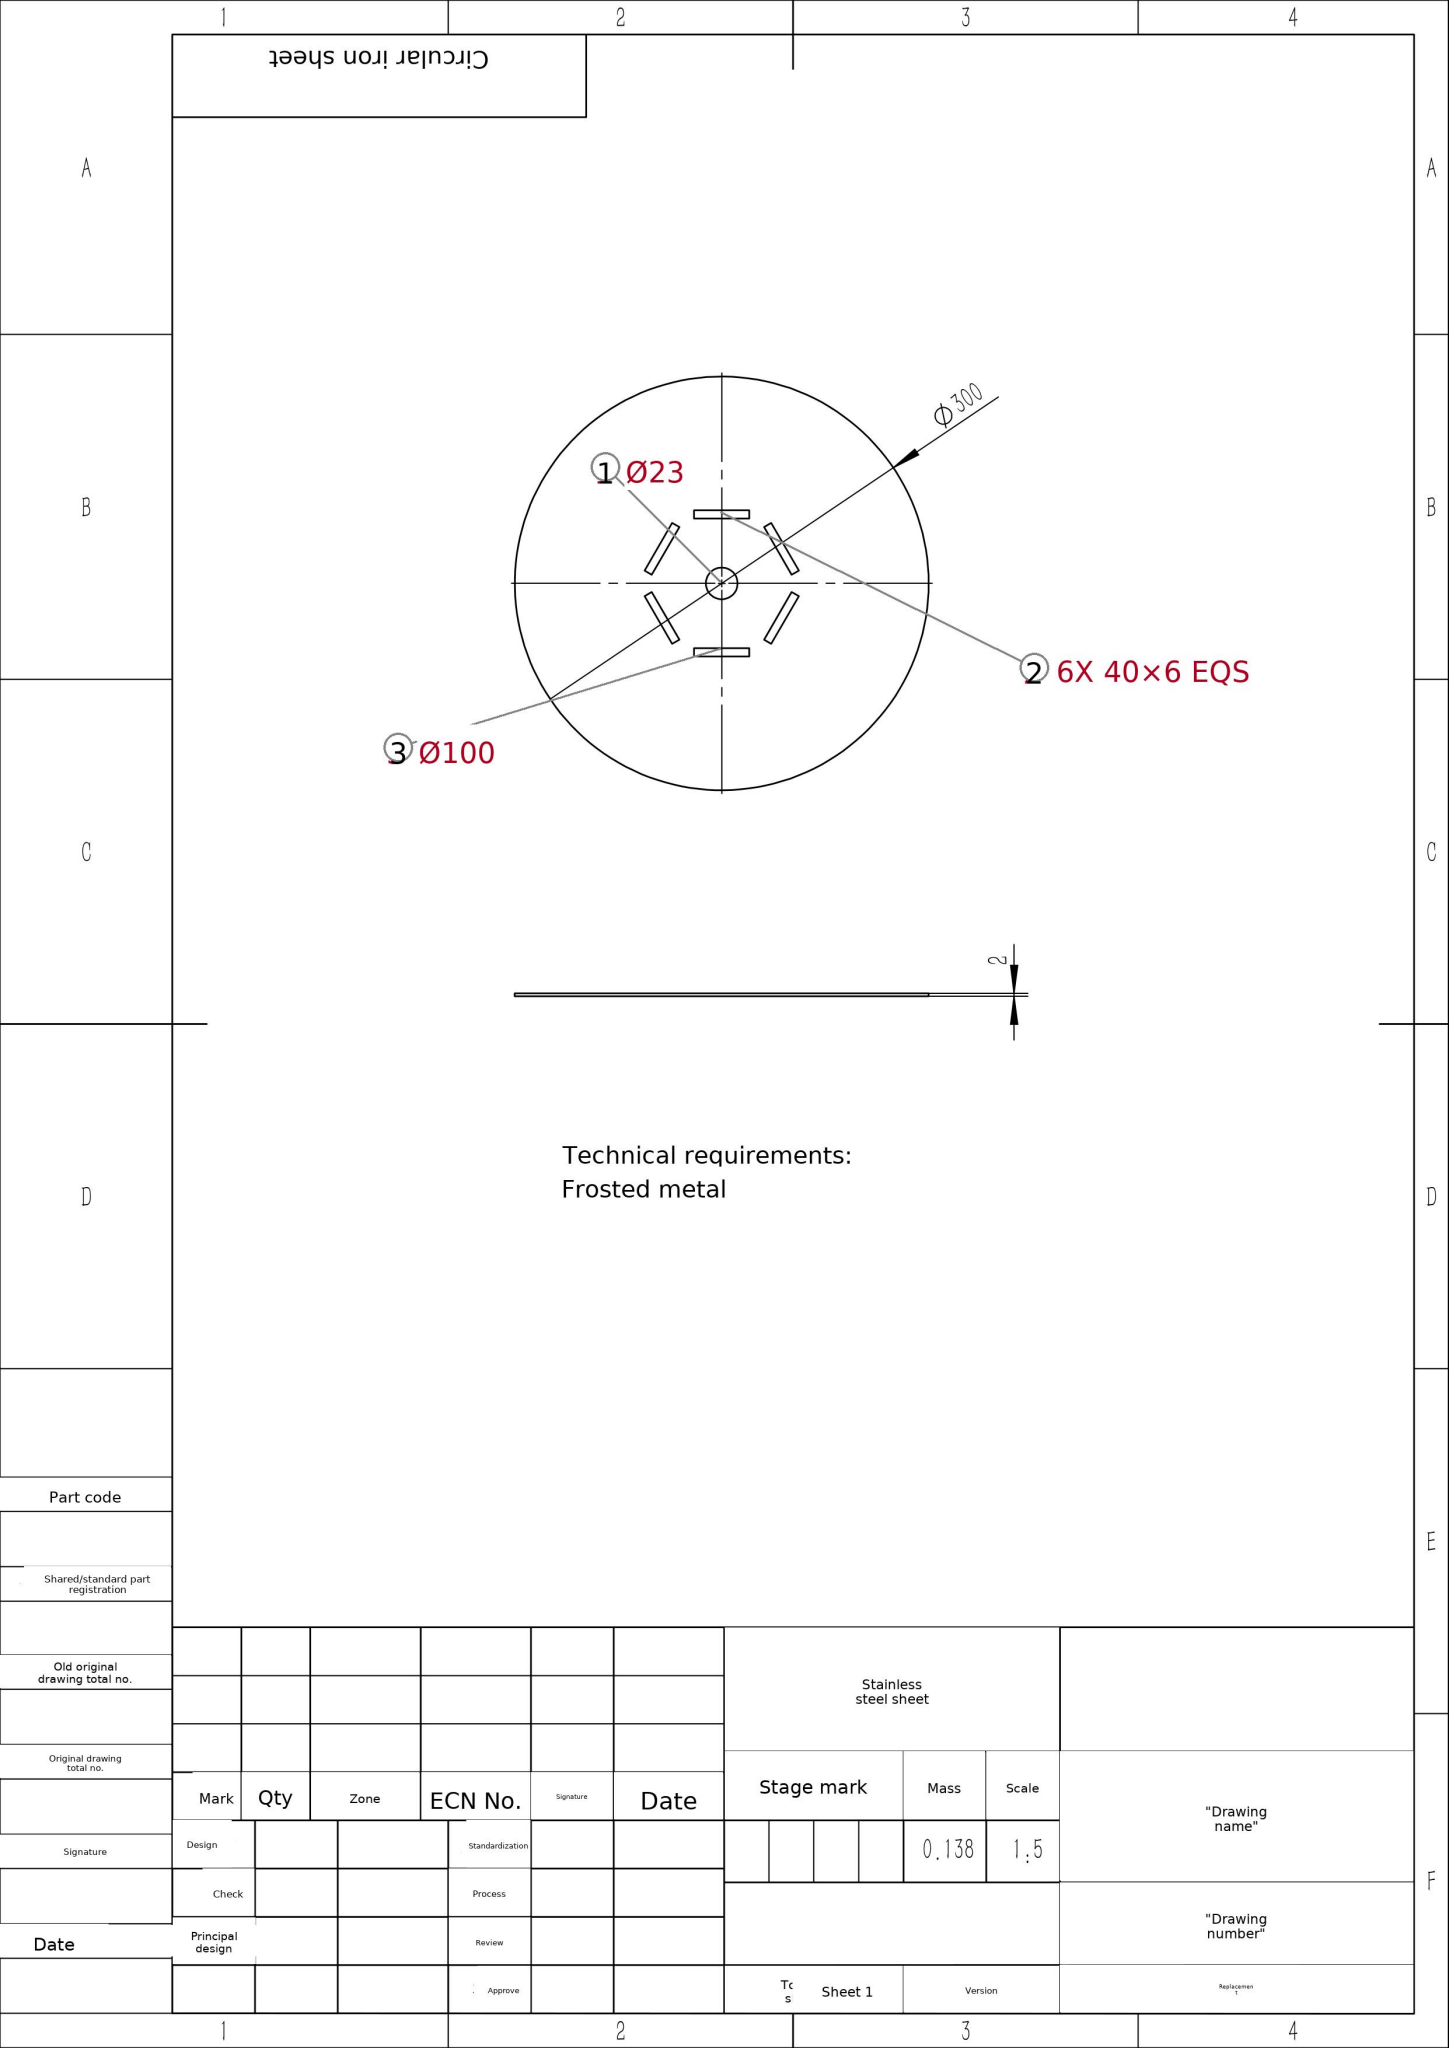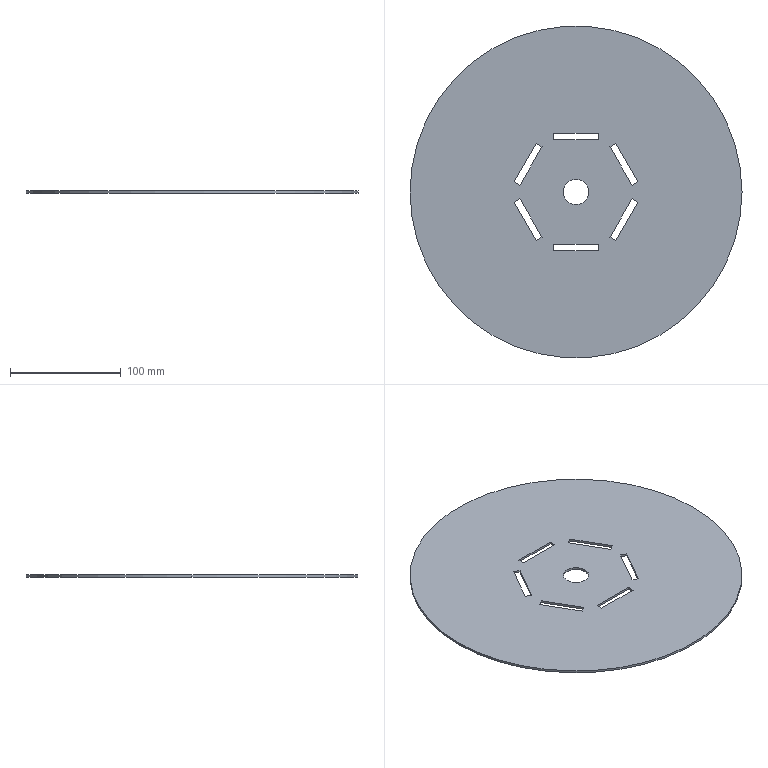Part | SolidWorks | mm | material Stainless steel sheet | 1 solid | 30 faces | box 300 x 300 x 2 mm | volume 137661 mm3 | plane 26 | cylinder 4 | commonest cylinder face diameters 23 x2 300 x2
build123d program:
from build123d import *

# Parameters (mm, degrees)
SKETCH1_R           = 150
SKETCH1_R_2         = 11.5
BOSS_EXTRUDE1_DEPTH = 2
SKETCH3_W           = 40
SKETCH3_H           = 6
CUT_EXTRUDE1_DEPTH  = 2
CIRPATTERN1_COUNT   = 6


with BuildPart() as part:
    # Sketch1 → Boss-Extrude1 (new body)
    with BuildSketch(Plane.XY):
        Circle(SKETCH1_R)
        Circle(SKETCH1_R_2, mode=Mode.SUBTRACT)
    extrude(amount=BOSS_EXTRUDE1_DEPTH)

    # Sketch3 → Cut-Extrude1 (cut)
    with BuildSketch(Plane.XY.offset(2)):
        with Locations((0, 50)):
            Rectangle(SKETCH3_W, SKETCH3_H)
    cut_extrude1 = extrude(amount=-CUT_EXTRUDE1_DEPTH, mode=Mode.SUBTRACT)

    # CirPattern1: Cut-Extrude1 ×6 about axis
    cirpattern1_axis = Axis((0, 0, 0), (0, 0, 1))
    for i in range(1, CIRPATTERN1_COUNT):
        add(cut_extrude1.rotate(cirpattern1_axis, i * 360 / CIRPATTERN1_COUNT), mode=Mode.SUBTRACT)


solid = part.part
STEP:
#1=CARTESIAN_POINT('',(-11.5,0.,2.));
#2=VERTEX_POINT('',#1);
#3=CARTESIAN_POINT('',(11.5,0.,2.));
#4=VERTEX_POINT('',#3);
#5=CARTESIAN_POINT('',(0.,0.,2.));
#6=DIRECTION('',(0.,0.,1.));
#7=DIRECTION('',(1.,0.,0.));
#8=AXIS2_PLACEMENT_3D('',#5,#6,#7);
#9=CIRCLE('',#8,11.5);
#10=EDGE_CURVE('',#2,#4,#9,.T.);
#11=ORIENTED_EDGE('',*,*,#10,.T.);
#12=CARTESIAN_POINT('',(11.5,0.,0.));
#13=VERTEX_POINT('',#12);
#14=CARTESIAN_POINT('',(11.5,0.,2.));
#15=DIRECTION('',(0.,0.,-1.));
#16=VECTOR('',#15,1000.);
#17=LINE('',#14,#16);
#18=EDGE_CURVE('',#4,#13,#17,.T.);
#19=ORIENTED_EDGE('',*,*,#18,.T.);
#20=CARTESIAN_POINT('',(-11.5,0.,0.));
#21=VERTEX_POINT('',#20);
#22=CARTESIAN_POINT('',(0.,0.,0.));
#23=DIRECTION('',(0.,0.,1.));
#24=DIRECTION('',(1.,0.,0.));
#25=AXIS2_PLACEMENT_3D('',#22,#23,#24);
#26=CIRCLE('',#25,11.5);
#27=EDGE_CURVE('',#21,#13,#26,.T.);
#28=ORIENTED_EDGE('',*,*,#27,.F.);
#29=CARTESIAN_POINT('',(-11.5,0.,2.));
#30=DIRECTION('',(0.,0.,-1.));
#31=VECTOR('',#30,1000.);
#32=LINE('',#29,#31);
#33=EDGE_CURVE('',#2,#21,#32,.T.);
#34=ORIENTED_EDGE('',*,*,#33,.F.);
#35=EDGE_LOOP('',(#11,#19,#28,#34));
#36=FACE_OUTER_BOUND('',#35,.T.);
#37=CARTESIAN_POINT('',(0.,0.,2.));
#38=DIRECTION('',(0.,0.,-1.));
#39=DIRECTION('',(-1.,0.,0.));
#40=AXIS2_PLACEMENT_3D('',#37,#38,#39);
#41=CYLINDRICAL_SURFACE('',#40,11.5);
#42=ADVANCED_FACE('',(#36),#41,.F.);
#43=CARTESIAN_POINT('',(150.,0.,2.));
#44=VERTEX_POINT('',#43);
#45=CARTESIAN_POINT('',(-150.,0.,2.));
#46=VERTEX_POINT('',#45);
#47=CARTESIAN_POINT('',(0.,0.,2.));
#48=DIRECTION('',(0.,0.,1.));
#49=DIRECTION('',(1.,0.,0.));
#50=AXIS2_PLACEMENT_3D('',#47,#48,#49);
#51=CIRCLE('',#50,150.);
#52=EDGE_CURVE('',#44,#46,#51,.T.);
#53=ORIENTED_EDGE('',*,*,#52,.F.);
#54=CARTESIAN_POINT('',(150.,0.,0.));
#55=VERTEX_POINT('',#54);
#56=CARTESIAN_POINT('',(150.,0.,2.));
#57=DIRECTION('',(0.,0.,-1.));
#58=VECTOR('',#57,1000.);
#59=LINE('',#56,#58);
#60=EDGE_CURVE('',#44,#55,#59,.T.);
#61=ORIENTED_EDGE('',*,*,#60,.T.);
#62=CARTESIAN_POINT('',(-150.,0.,0.));
#63=VERTEX_POINT('',#62);
#64=CARTESIAN_POINT('',(0.,0.,0.));
#65=DIRECTION('',(0.,0.,1.));
#66=DIRECTION('',(1.,0.,0.));
#67=AXIS2_PLACEMENT_3D('',#64,#65,#66);
#68=CIRCLE('',#67,150.);
#69=EDGE_CURVE('',#55,#63,#68,.T.);
#70=ORIENTED_EDGE('',*,*,#69,.T.);
#71=CARTESIAN_POINT('',(-150.,0.,2.));
#72=DIRECTION('',(0.,0.,-1.));
#73=VECTOR('',#72,1000.);
#74=LINE('',#71,#73);
#75=EDGE_CURVE('',#46,#63,#74,.T.);
#76=ORIENTED_EDGE('',*,*,#75,.F.);
#77=EDGE_LOOP('',(#53,#61,#70,#76));
#78=FACE_OUTER_BOUND('',#77,.T.);
#79=CARTESIAN_POINT('',(0.,0.,2.));
#80=DIRECTION('',(0.,0.,-1.));
#81=DIRECTION('',(-1.,0.,0.));
#82=AXIS2_PLACEMENT_3D('',#79,#80,#81);
#83=CYLINDRICAL_SURFACE('',#82,150.);
#84=ADVANCED_FACE('',(#78),#83,.T.);
#85=CARTESIAN_POINT('',(-55.899,9.179,2.));
#86=VERTEX_POINT('',#85);
#87=CARTESIAN_POINT('',(-50.703,6.179,2.));
#88=VERTEX_POINT('',#87);
#89=CARTESIAN_POINT('',(-50.703,6.179,2.));
#90=DIRECTION('',(0.866,-0.5,0.));
#91=VECTOR('',#90,1000.);
#92=LINE('',#89,#91);
#93=EDGE_CURVE('',#86,#88,#92,.T.);
#94=ORIENTED_EDGE('',*,*,#93,.F.);
#95=CARTESIAN_POINT('',(-35.899,43.821,2.));
#96=VERTEX_POINT('',#95);
#97=CARTESIAN_POINT('',(-35.899,43.821,2.));
#98=DIRECTION('',(-0.5,-0.866,0.));
#99=VECTOR('',#98,1000.);
#100=LINE('',#97,#99);
#101=EDGE_CURVE('',#96,#86,#100,.T.);
#102=ORIENTED_EDGE('',*,*,#101,.F.);
#103=CARTESIAN_POINT('',(-30.703,40.821,2.));
#104=VERTEX_POINT('',#103);
#105=CARTESIAN_POINT('',(-30.703,40.821,2.));
#106=DIRECTION('',(-0.866,0.5,0.));
#107=VECTOR('',#106,1000.);
#108=LINE('',#105,#107);
#109=EDGE_CURVE('',#104,#96,#108,.T.);
#110=ORIENTED_EDGE('',*,*,#109,.F.);
#111=CARTESIAN_POINT('',(-30.703,40.821,2.));
#112=DIRECTION('',(0.5,0.866,0.));
#113=VECTOR('',#112,1000.);
#114=LINE('',#111,#113);
#115=EDGE_CURVE('',#88,#104,#114,.T.);
#116=ORIENTED_EDGE('',*,*,#115,.F.);
#117=EDGE_LOOP('',(#94,#102,#110,#116));
#118=FACE_BOUND('',#117,.T.);
#119=CARTESIAN_POINT('',(-35.899,-43.821,2.));
#120=VERTEX_POINT('',#119);
#121=CARTESIAN_POINT('',(-30.703,-40.821,2.));
#122=VERTEX_POINT('',#121);
#123=CARTESIAN_POINT('',(-30.703,-40.821,2.));
#124=DIRECTION('',(0.866,0.5,0.));
#125=VECTOR('',#124,1000.);
#126=LINE('',#123,#125);
#127=EDGE_CURVE('',#120,#122,#126,.T.);
#128=ORIENTED_EDGE('',*,*,#127,.F.);
#129=CARTESIAN_POINT('',(-55.899,-9.179,2.));
#130=VERTEX_POINT('',#129);
#131=CARTESIAN_POINT('',(-55.899,-9.179,2.));
#132=DIRECTION('',(0.5,-0.866,0.));
#133=VECTOR('',#132,1000.);
#134=LINE('',#131,#133);
#135=EDGE_CURVE('',#130,#120,#134,.T.);
#136=ORIENTED_EDGE('',*,*,#135,.F.);
#137=CARTESIAN_POINT('',(-50.703,-6.179,2.));
#138=VERTEX_POINT('',#137);
#139=CARTESIAN_POINT('',(-50.703,-6.179,2.));
#140=DIRECTION('',(-0.866,-0.5,0.));
#141=VECTOR('',#140,1000.);
#142=LINE('',#139,#141);
#143=EDGE_CURVE('',#138,#130,#142,.T.);
#144=ORIENTED_EDGE('',*,*,#143,.F.);
#145=CARTESIAN_POINT('',(-50.703,-6.179,2.));
#146=DIRECTION('',(-0.5,0.866,0.));
#147=VECTOR('',#146,1000.);
#148=LINE('',#145,#147);
#149=EDGE_CURVE('',#122,#138,#148,.T.);
#150=ORIENTED_EDGE('',*,*,#149,.F.);
#151=EDGE_LOOP('',(#128,#136,#144,#150));
#152=FACE_BOUND('',#151,.T.);
#153=CARTESIAN_POINT('',(20.,-53.,2.));
#154=VERTEX_POINT('',#153);
#155=CARTESIAN_POINT('',(20.,-47.,2.));
#156=VERTEX_POINT('',#155);
#157=CARTESIAN_POINT('',(20.,-47.,2.));
#158=DIRECTION('',(0.,1.,0.));
#159=VECTOR('',#158,1000.);
#160=LINE('',#157,#159);
#161=EDGE_CURVE('',#154,#156,#160,.T.);
#162=ORIENTED_EDGE('',*,*,#161,.F.);
#163=CARTESIAN_POINT('',(-20.,-53.,2.));
#164=VERTEX_POINT('',#163);
#165=CARTESIAN_POINT('',(-20.,-53.,2.));
#166=DIRECTION('',(1.,0.,0.));
#167=VECTOR('',#166,1000.);
#168=LINE('',#165,#167);
#169=EDGE_CURVE('',#164,#154,#168,.T.);
#170=ORIENTED_EDGE('',*,*,#169,.F.);
#171=CARTESIAN_POINT('',(-20.,-47.,2.));
#172=VERTEX_POINT('',#171);
#173=CARTESIAN_POINT('',(-20.,-47.,2.));
#174=DIRECTION('',(0.,-1.,0.));
#175=VECTOR('',#174,1000.);
#176=LINE('',#173,#175);
#177=EDGE_CURVE('',#172,#164,#176,.T.);
#178=ORIENTED_EDGE('',*,*,#177,.F.);
#179=CARTESIAN_POINT('',(-20.,-47.,2.));
#180=DIRECTION('',(-1.,-0.,0.));
#181=VECTOR('',#180,1000.);
#182=LINE('',#179,#181);
#183=EDGE_CURVE('',#156,#172,#182,.T.);
#184=ORIENTED_EDGE('',*,*,#183,.F.);
#185=EDGE_LOOP('',(#162,#170,#178,#184));
#186=FACE_BOUND('',#185,.T.);
#187=CARTESIAN_POINT('',(55.899,-9.179,2.));
#188=VERTEX_POINT('',#187);
#189=CARTESIAN_POINT('',(50.703,-6.179,2.));
#190=VERTEX_POINT('',#189);
#191=CARTESIAN_POINT('',(50.703,-6.179,2.));
#192=DIRECTION('',(-0.866,0.5,0.));
#193=VECTOR('',#192,1000.);
#194=LINE('',#191,#193);
#195=EDGE_CURVE('',#188,#190,#194,.T.);
#196=ORIENTED_EDGE('',*,*,#195,.F.);
#197=CARTESIAN_POINT('',(35.899,-43.821,2.));
#198=VERTEX_POINT('',#197);
#199=CARTESIAN_POINT('',(35.899,-43.821,2.));
#200=DIRECTION('',(0.5,0.866,0.));
#201=VECTOR('',#200,1000.);
#202=LINE('',#199,#201);
#203=EDGE_CURVE('',#198,#188,#202,.T.);
#204=ORIENTED_EDGE('',*,*,#203,.F.);
#205=CARTESIAN_POINT('',(30.703,-40.821,2.));
#206=VERTEX_POINT('',#205);
#207=CARTESIAN_POINT('',(30.703,-40.821,2.));
#208=DIRECTION('',(0.866,-0.5,0.));
#209=VECTOR('',#208,1000.);
#210=LINE('',#207,#209);
#211=EDGE_CURVE('',#206,#198,#210,.T.);
#212=ORIENTED_EDGE('',*,*,#211,.F.);
#213=CARTESIAN_POINT('',(30.703,-40.821,2.));
#214=DIRECTION('',(-0.5,-0.866,0.));
#215=VECTOR('',#214,1000.);
#216=LINE('',#213,#215);
#217=EDGE_CURVE('',#190,#206,#216,.T.);
#218=ORIENTED_EDGE('',*,*,#217,.F.);
#219=EDGE_LOOP('',(#196,#204,#212,#218));
#220=FACE_BOUND('',#219,.T.);
#221=CARTESIAN_POINT('',(35.899,43.821,2.));
#222=VERTEX_POINT('',#221);
#223=CARTESIAN_POINT('',(30.703,40.821,2.));
#224=VERTEX_POINT('',#223);
#225=CARTESIAN_POINT('',(30.703,40.821,2.));
#226=DIRECTION('',(-0.866,-0.5,0.));
#227=VECTOR('',#226,1000.);
#228=LINE('',#225,#227);
#229=EDGE_CURVE('',#222,#224,#228,.T.);
#230=ORIENTED_EDGE('',*,*,#229,.F.);
#231=CARTESIAN_POINT('',(55.899,9.179,2.));
#232=VERTEX_POINT('',#231);
#233=CARTESIAN_POINT('',(55.899,9.179,2.));
#234=DIRECTION('',(-0.5,0.866,0.));
#235=VECTOR('',#234,1000.);
#236=LINE('',#233,#235);
#237=EDGE_CURVE('',#232,#222,#236,.T.);
#238=ORIENTED_EDGE('',*,*,#237,.F.);
#239=CARTESIAN_POINT('',(50.703,6.179,2.));
#240=VERTEX_POINT('',#239);
#241=CARTESIAN_POINT('',(50.703,6.179,2.));
#242=DIRECTION('',(0.866,0.5,0.));
#243=VECTOR('',#242,1000.);
#244=LINE('',#241,#243);
#245=EDGE_CURVE('',#240,#232,#244,.T.);
#246=ORIENTED_EDGE('',*,*,#245,.F.);
#247=CARTESIAN_POINT('',(50.703,6.179,2.));
#248=DIRECTION('',(0.5,-0.866,0.));
#249=VECTOR('',#248,1000.);
#250=LINE('',#247,#249);
#251=EDGE_CURVE('',#224,#240,#250,.T.);
#252=ORIENTED_EDGE('',*,*,#251,.F.);
#253=EDGE_LOOP('',(#230,#238,#246,#252));
#254=FACE_BOUND('',#253,.T.);
#255=CARTESIAN_POINT('',(-20.,53.,2.));
#256=VERTEX_POINT('',#255);
#257=CARTESIAN_POINT('',(-20.,47.,2.));
#258=VERTEX_POINT('',#257);
#259=CARTESIAN_POINT('',(-20.,47.,2.));
#260=DIRECTION('',(0.,-1.,0.));
#261=VECTOR('',#260,1000.);
#262=LINE('',#259,#261);
#263=EDGE_CURVE('',#256,#258,#262,.T.);
#264=ORIENTED_EDGE('',*,*,#263,.F.);
#265=CARTESIAN_POINT('',(20.,53.,2.));
#266=VERTEX_POINT('',#265);
#267=CARTESIAN_POINT('',(20.,53.,2.));
#268=DIRECTION('',(-1.,0.,0.));
#269=VECTOR('',#268,1000.);
#270=LINE('',#267,#269);
#271=EDGE_CURVE('',#266,#256,#270,.T.);
#272=ORIENTED_EDGE('',*,*,#271,.F.);
#273=CARTESIAN_POINT('',(20.,47.,2.));
#274=VERTEX_POINT('',#273);
#275=CARTESIAN_POINT('',(20.,47.,2.));
#276=DIRECTION('',(0.,1.,0.));
#277=VECTOR('',#276,1000.);
#278=LINE('',#275,#277);
#279=EDGE_CURVE('',#274,#266,#278,.T.);
#280=ORIENTED_EDGE('',*,*,#279,.F.);
#281=CARTESIAN_POINT('',(20.,47.,2.));
#282=DIRECTION('',(1.,0.,0.));
#283=VECTOR('',#282,1000.);
#284=LINE('',#281,#283);
#285=EDGE_CURVE('',#258,#274,#284,.T.);
#286=ORIENTED_EDGE('',*,*,#285,.F.);
#287=EDGE_LOOP('',(#264,#272,#280,#286));
#288=FACE_BOUND('',#287,.T.);
#289=CARTESIAN_POINT('',(0.,0.,2.));
#290=DIRECTION('',(0.,0.,1.));
#291=DIRECTION('',(1.,0.,0.));
#292=AXIS2_PLACEMENT_3D('',#289,#290,#291);
#293=CIRCLE('',#292,150.);
#294=EDGE_CURVE('',#46,#44,#293,.T.);
#295=ORIENTED_EDGE('',*,*,#294,.T.);
#296=ORIENTED_EDGE('',*,*,#52,.T.);
#297=EDGE_LOOP('',(#295,#296));
#298=FACE_OUTER_BOUND('',#297,.T.);
#299=ORIENTED_EDGE('',*,*,#10,.F.);
#300=CARTESIAN_POINT('',(0.,0.,2.));
#301=DIRECTION('',(0.,0.,1.));
#302=DIRECTION('',(1.,0.,0.));
#303=AXIS2_PLACEMENT_3D('',#300,#301,#302);
#304=CIRCLE('',#303,11.5);
#305=EDGE_CURVE('',#4,#2,#304,.T.);
#306=ORIENTED_EDGE('',*,*,#305,.F.);
#307=EDGE_LOOP('',(#299,#306));
#308=FACE_BOUND('',#307,.T.);
#309=CARTESIAN_POINT('',(0.,0.,2.));
#310=DIRECTION('',(0.,0.,1.));
#311=DIRECTION('',(1.,0.,0.));
#312=AXIS2_PLACEMENT_3D('',#309,#310,#311);
#313=PLANE('',#312);
#314=ADVANCED_FACE('',(#118,#152,#186,#220,#254,#288,#298,#308),#313,.T.);
#315=CARTESIAN_POINT('',(-35.899,43.821,0.));
#316=VERTEX_POINT('',#315);
#317=CARTESIAN_POINT('',(-55.899,9.179,0.));
#318=VERTEX_POINT('',#317);
#319=CARTESIAN_POINT('',(-35.899,43.821,0.));
#320=DIRECTION('',(-0.5,-0.866,0.));
#321=VECTOR('',#320,1000.);
#322=LINE('',#319,#321);
#323=EDGE_CURVE('',#316,#318,#322,.T.);
#324=ORIENTED_EDGE('',*,*,#323,.T.);
#325=CARTESIAN_POINT('',(-50.703,6.179,0.));
#326=VERTEX_POINT('',#325);
#327=CARTESIAN_POINT('',(-50.703,6.179,0.));
#328=DIRECTION('',(0.866,-0.5,0.));
#329=VECTOR('',#328,1000.);
#330=LINE('',#327,#329);
#331=EDGE_CURVE('',#318,#326,#330,.T.);
#332=ORIENTED_EDGE('',*,*,#331,.T.);
#333=CARTESIAN_POINT('',(-30.703,40.821,0.));
#334=VERTEX_POINT('',#333);
#335=CARTESIAN_POINT('',(-30.703,40.821,0.));
#336=DIRECTION('',(0.5,0.866,0.));
#337=VECTOR('',#336,1000.);
#338=LINE('',#335,#337);
#339=EDGE_CURVE('',#326,#334,#338,.T.);
#340=ORIENTED_EDGE('',*,*,#339,.T.);
#341=CARTESIAN_POINT('',(-30.703,40.821,0.));
#342=DIRECTION('',(-0.866,0.5,0.));
#343=VECTOR('',#342,1000.);
#344=LINE('',#341,#343);
#345=EDGE_CURVE('',#334,#316,#344,.T.);
#346=ORIENTED_EDGE('',*,*,#345,.T.);
#347=EDGE_LOOP('',(#324,#332,#340,#346));
#348=FACE_BOUND('',#347,.T.);
#349=CARTESIAN_POINT('',(-55.899,-9.179,0.));
#350=VERTEX_POINT('',#349);
#351=CARTESIAN_POINT('',(-35.899,-43.821,0.));
#352=VERTEX_POINT('',#351);
#353=CARTESIAN_POINT('',(-55.899,-9.179,0.));
#354=DIRECTION('',(0.5,-0.866,0.));
#355=VECTOR('',#354,1000.);
#356=LINE('',#353,#355);
#357=EDGE_CURVE('',#350,#352,#356,.T.);
#358=ORIENTED_EDGE('',*,*,#357,.T.);
#359=CARTESIAN_POINT('',(-30.703,-40.821,0.));
#360=VERTEX_POINT('',#359);
#361=CARTESIAN_POINT('',(-30.703,-40.821,0.));
#362=DIRECTION('',(0.866,0.5,0.));
#363=VECTOR('',#362,1000.);
#364=LINE('',#361,#363);
#365=EDGE_CURVE('',#352,#360,#364,.T.);
#366=ORIENTED_EDGE('',*,*,#365,.T.);
#367=CARTESIAN_POINT('',(-50.703,-6.179,0.));
#368=VERTEX_POINT('',#367);
#369=CARTESIAN_POINT('',(-50.703,-6.179,0.));
#370=DIRECTION('',(-0.5,0.866,0.));
#371=VECTOR('',#370,1000.);
#372=LINE('',#369,#371);
#373=EDGE_CURVE('',#360,#368,#372,.T.);
#374=ORIENTED_EDGE('',*,*,#373,.T.);
#375=CARTESIAN_POINT('',(-50.703,-6.179,0.));
#376=DIRECTION('',(-0.866,-0.5,0.));
#377=VECTOR('',#376,1000.);
#378=LINE('',#375,#377);
#379=EDGE_CURVE('',#368,#350,#378,.T.);
#380=ORIENTED_EDGE('',*,*,#379,.T.);
#381=EDGE_LOOP('',(#358,#366,#374,#380));
#382=FACE_BOUND('',#381,.T.);
#383=CARTESIAN_POINT('',(-20.,-53.,0.));
#384=VERTEX_POINT('',#383);
#385=CARTESIAN_POINT('',(20.,-53.,0.));
#386=VERTEX_POINT('',#385);
#387=CARTESIAN_POINT('',(-20.,-53.,0.));
#388=DIRECTION('',(1.,0.,0.));
#389=VECTOR('',#388,1000.);
#390=LINE('',#387,#389);
#391=EDGE_CURVE('',#384,#386,#390,.T.);
#392=ORIENTED_EDGE('',*,*,#391,.T.);
#393=CARTESIAN_POINT('',(20.,-47.,0.));
#394=VERTEX_POINT('',#393);
#395=CARTESIAN_POINT('',(20.,-47.,0.));
#396=DIRECTION('',(0.,1.,0.));
#397=VECTOR('',#396,1000.);
#398=LINE('',#395,#397);
#399=EDGE_CURVE('',#386,#394,#398,.T.);
#400=ORIENTED_EDGE('',*,*,#399,.T.);
#401=CARTESIAN_POINT('',(-20.,-47.,0.));
#402=VERTEX_POINT('',#401);
#403=CARTESIAN_POINT('',(-20.,-47.,0.));
#404=DIRECTION('',(-1.,-0.,0.));
#405=VECTOR('',#404,1000.);
#406=LINE('',#403,#405);
#407=EDGE_CURVE('',#394,#402,#406,.T.);
#408=ORIENTED_EDGE('',*,*,#407,.T.);
#409=CARTESIAN_POINT('',(-20.,-47.,0.));
#410=DIRECTION('',(0.,-1.,0.));
#411=VECTOR('',#410,1000.);
#412=LINE('',#409,#411);
#413=EDGE_CURVE('',#402,#384,#412,.T.);
#414=ORIENTED_EDGE('',*,*,#413,.T.);
#415=EDGE_LOOP('',(#392,#400,#408,#414));
#416=FACE_BOUND('',#415,.T.);
#417=CARTESIAN_POINT('',(35.899,-43.821,0.));
#418=VERTEX_POINT('',#417);
#419=CARTESIAN_POINT('',(55.899,-9.179,0.));
#420=VERTEX_POINT('',#419);
#421=CARTESIAN_POINT('',(35.899,-43.821,0.));
#422=DIRECTION('',(0.5,0.866,0.));
#423=VECTOR('',#422,1000.);
#424=LINE('',#421,#423);
#425=EDGE_CURVE('',#418,#420,#424,.T.);
#426=ORIENTED_EDGE('',*,*,#425,.T.);
#427=CARTESIAN_POINT('',(50.703,-6.179,0.));
#428=VERTEX_POINT('',#427);
#429=CARTESIAN_POINT('',(50.703,-6.179,0.));
#430=DIRECTION('',(-0.866,0.5,0.));
#431=VECTOR('',#430,1000.);
#432=LINE('',#429,#431);
#433=EDGE_CURVE('',#420,#428,#432,.T.);
#434=ORIENTED_EDGE('',*,*,#433,.T.);
#435=CARTESIAN_POINT('',(30.703,-40.821,0.));
#436=VERTEX_POINT('',#435);
#437=CARTESIAN_POINT('',(30.703,-40.821,0.));
#438=DIRECTION('',(-0.5,-0.866,0.));
#439=VECTOR('',#438,1000.);
#440=LINE('',#437,#439);
#441=EDGE_CURVE('',#428,#436,#440,.T.);
#442=ORIENTED_EDGE('',*,*,#441,.T.);
#443=CARTESIAN_POINT('',(30.703,-40.821,0.));
#444=DIRECTION('',(0.866,-0.5,0.));
#445=VECTOR('',#444,1000.);
#446=LINE('',#443,#445);
#447=EDGE_CURVE('',#436,#418,#446,.T.);
#448=ORIENTED_EDGE('',*,*,#447,.T.);
#449=EDGE_LOOP('',(#426,#434,#442,#448));
#450=FACE_BOUND('',#449,.T.);
#451=CARTESIAN_POINT('',(55.899,9.179,0.));
#452=VERTEX_POINT('',#451);
#453=CARTESIAN_POINT('',(35.899,43.821,0.));
#454=VERTEX_POINT('',#453);
#455=CARTESIAN_POINT('',(55.899,9.179,0.));
#456=DIRECTION('',(-0.5,0.866,0.));
#457=VECTOR('',#456,1000.);
#458=LINE('',#455,#457);
#459=EDGE_CURVE('',#452,#454,#458,.T.);
#460=ORIENTED_EDGE('',*,*,#459,.T.);
#461=CARTESIAN_POINT('',(30.703,40.821,0.));
#462=VERTEX_POINT('',#461);
#463=CARTESIAN_POINT('',(30.703,40.821,0.));
#464=DIRECTION('',(-0.866,-0.5,0.));
#465=VECTOR('',#464,1000.);
#466=LINE('',#463,#465);
#467=EDGE_CURVE('',#454,#462,#466,.T.);
#468=ORIENTED_EDGE('',*,*,#467,.T.);
#469=CARTESIAN_POINT('',(50.703,6.179,0.));
#470=VERTEX_POINT('',#469);
#471=CARTESIAN_POINT('',(50.703,6.179,0.));
#472=DIRECTION('',(0.5,-0.866,0.));
#473=VECTOR('',#472,1000.);
#474=LINE('',#471,#473);
#475=EDGE_CURVE('',#462,#470,#474,.T.);
#476=ORIENTED_EDGE('',*,*,#475,.T.);
#477=CARTESIAN_POINT('',(50.703,6.179,0.));
#478=DIRECTION('',(0.866,0.5,0.));
#479=VECTOR('',#478,1000.);
#480=LINE('',#477,#479);
#481=EDGE_CURVE('',#470,#452,#480,.T.);
#482=ORIENTED_EDGE('',*,*,#481,.T.);
#483=EDGE_LOOP('',(#460,#468,#476,#482));
#484=FACE_BOUND('',#483,.T.);
#485=CARTESIAN_POINT('',(20.,53.,0.));
#486=VERTEX_POINT('',#485);
#487=CARTESIAN_POINT('',(-20.,53.,0.));
#488=VERTEX_POINT('',#487);
#489=CARTESIAN_POINT('',(20.,53.,0.));
#490=DIRECTION('',(-1.,0.,0.));
#491=VECTOR('',#490,1000.);
#492=LINE('',#489,#491);
#493=EDGE_CURVE('',#486,#488,#492,.T.);
#494=ORIENTED_EDGE('',*,*,#493,.T.);
#495=CARTESIAN_POINT('',(-20.,47.,0.));
#496=VERTEX_POINT('',#495);
#497=CARTESIAN_POINT('',(-20.,47.,0.));
#498=DIRECTION('',(0.,-1.,0.));
#499=VECTOR('',#498,1000.);
#500=LINE('',#497,#499);
#501=EDGE_CURVE('',#488,#496,#500,.T.);
#502=ORIENTED_EDGE('',*,*,#501,.T.);
#503=CARTESIAN_POINT('',(20.,47.,0.));
#504=VERTEX_POINT('',#503);
#505=CARTESIAN_POINT('',(20.,47.,0.));
#506=DIRECTION('',(1.,0.,0.));
#507=VECTOR('',#506,1000.);
#508=LINE('',#505,#507);
#509=EDGE_CURVE('',#496,#504,#508,.T.);
#510=ORIENTED_EDGE('',*,*,#509,.T.);
#511=CARTESIAN_POINT('',(20.,47.,0.));
#512=DIRECTION('',(0.,1.,0.));
#513=VECTOR('',#512,1000.);
#514=LINE('',#511,#513);
#515=EDGE_CURVE('',#504,#486,#514,.T.);
#516=ORIENTED_EDGE('',*,*,#515,.T.);
#517=EDGE_LOOP('',(#494,#502,#510,#516));
#518=FACE_BOUND('',#517,.T.);
#519=CARTESIAN_POINT('',(0.,0.,0.));
#520=DIRECTION('',(0.,0.,1.));
#521=DIRECTION('',(1.,0.,0.));
#522=AXIS2_PLACEMENT_3D('',#519,#520,#521);
#523=CIRCLE('',#522,150.);
#524=EDGE_CURVE('',#63,#55,#523,.T.);
#525=ORIENTED_EDGE('',*,*,#524,.F.);
#526=ORIENTED_EDGE('',*,*,#69,.F.);
#527=EDGE_LOOP('',(#525,#526));
#528=FACE_OUTER_BOUND('',#527,.T.);
#529=ORIENTED_EDGE('',*,*,#27,.T.);
#530=CARTESIAN_POINT('',(0.,0.,0.));
#531=DIRECTION('',(0.,0.,1.));
#532=DIRECTION('',(1.,0.,0.));
#533=AXIS2_PLACEMENT_3D('',#530,#531,#532);
#534=CIRCLE('',#533,11.5);
#535=EDGE_CURVE('',#13,#21,#534,.T.);
#536=ORIENTED_EDGE('',*,*,#535,.T.);
#537=EDGE_LOOP('',(#529,#536));
#538=FACE_BOUND('',#537,.T.);
#539=CARTESIAN_POINT('',(0.,0.,0.));
#540=DIRECTION('',(0.,0.,1.));
#541=DIRECTION('',(1.,0.,0.));
#542=AXIS2_PLACEMENT_3D('',#539,#540,#541);
#543=PLANE('',#542);
#544=ADVANCED_FACE('',(#348,#382,#416,#450,#484,#518,#528,#538),#543,.F.);
#545=ORIENTED_EDGE('',*,*,#60,.F.);
#546=ORIENTED_EDGE('',*,*,#294,.F.);
#547=ORIENTED_EDGE('',*,*,#75,.T.);
#548=ORIENTED_EDGE('',*,*,#524,.T.);
#549=EDGE_LOOP('',(#545,#546,#547,#548));
#550=FACE_OUTER_BOUND('',#549,.T.);
#551=CARTESIAN_POINT('',(0.,0.,2.));
#552=DIRECTION('',(0.,0.,-1.));
#553=DIRECTION('',(-1.,0.,0.));
#554=AXIS2_PLACEMENT_3D('',#551,#552,#553);
#555=CYLINDRICAL_SURFACE('',#554,150.);
#556=ADVANCED_FACE('',(#550),#555,.T.);
#557=ORIENTED_EDGE('',*,*,#18,.F.);
#558=ORIENTED_EDGE('',*,*,#305,.T.);
#559=ORIENTED_EDGE('',*,*,#33,.T.);
#560=ORIENTED_EDGE('',*,*,#535,.F.);
#561=EDGE_LOOP('',(#557,#558,#559,#560));
#562=FACE_OUTER_BOUND('',#561,.T.);
#563=CARTESIAN_POINT('',(0.,0.,2.));
#564=DIRECTION('',(0.,0.,-1.));
#565=DIRECTION('',(-1.,0.,0.));
#566=AXIS2_PLACEMENT_3D('',#563,#564,#565);
#567=CYLINDRICAL_SURFACE('',#566,11.5);
#568=ADVANCED_FACE('',(#562),#567,.F.);
#569=ORIENTED_EDGE('',*,*,#263,.T.);
#570=CARTESIAN_POINT('',(-20.,47.,0.));
#571=DIRECTION('',(0.,0.,1.));
#572=VECTOR('',#571,1000.);
#573=LINE('',#570,#572);
#574=EDGE_CURVE('',#496,#258,#573,.T.);
#575=ORIENTED_EDGE('',*,*,#574,.F.);
#576=ORIENTED_EDGE('',*,*,#501,.F.);
#577=CARTESIAN_POINT('',(-20.,53.,0.));
#578=DIRECTION('',(0.,0.,1.));
#579=VECTOR('',#578,1000.);
#580=LINE('',#577,#579);
#581=EDGE_CURVE('',#488,#256,#580,.T.);
#582=ORIENTED_EDGE('',*,*,#581,.T.);
#583=EDGE_LOOP('',(#569,#575,#576,#582));
#584=FACE_OUTER_BOUND('',#583,.T.);
#585=CARTESIAN_POINT('',(-20.,47.,0.));
#586=DIRECTION('',(-1.,0.,0.));
#587=DIRECTION('',(0.,0.,1.));
#588=AXIS2_PLACEMENT_3D('',#585,#586,#587);
#589=PLANE('',#588);
#590=ADVANCED_FACE('',(#584),#589,.F.);
#591=ORIENTED_EDGE('',*,*,#271,.T.);
#592=ORIENTED_EDGE('',*,*,#581,.F.);
#593=ORIENTED_EDGE('',*,*,#493,.F.);
#594=CARTESIAN_POINT('',(20.,53.,0.));
#595=DIRECTION('',(0.,0.,1.));
#596=VECTOR('',#595,1000.);
#597=LINE('',#594,#596);
#598=EDGE_CURVE('',#486,#266,#597,.T.);
#599=ORIENTED_EDGE('',*,*,#598,.T.);
#600=EDGE_LOOP('',(#591,#592,#593,#599));
#601=FACE_OUTER_BOUND('',#600,.T.);
#602=CARTESIAN_POINT('',(20.,53.,0.));
#603=DIRECTION('',(0.,1.,0.));
#604=DIRECTION('',(0.,0.,1.));
#605=AXIS2_PLACEMENT_3D('',#602,#603,#604);
#606=PLANE('',#605);
#607=ADVANCED_FACE('',(#601),#606,.F.);
#608=ORIENTED_EDGE('',*,*,#279,.T.);
#609=ORIENTED_EDGE('',*,*,#598,.F.);
#610=ORIENTED_EDGE('',*,*,#515,.F.);
#611=CARTESIAN_POINT('',(20.,47.,0.));
#612=DIRECTION('',(0.,0.,1.));
#613=VECTOR('',#612,1000.);
#614=LINE('',#611,#613);
#615=EDGE_CURVE('',#504,#274,#614,.T.);
#616=ORIENTED_EDGE('',*,*,#615,.T.);
#617=EDGE_LOOP('',(#608,#609,#610,#616));
#618=FACE_OUTER_BOUND('',#617,.T.);
#619=CARTESIAN_POINT('',(20.,47.,0.));
#620=DIRECTION('',(1.,0.,0.));
#621=DIRECTION('',(0.,0.,-1.));
#622=AXIS2_PLACEMENT_3D('',#619,#620,#621);
#623=PLANE('',#622);
#624=ADVANCED_FACE('',(#618),#623,.F.);
#625=ORIENTED_EDGE('',*,*,#285,.T.);
#626=ORIENTED_EDGE('',*,*,#615,.F.);
#627=ORIENTED_EDGE('',*,*,#509,.F.);
#628=ORIENTED_EDGE('',*,*,#574,.T.);
#629=EDGE_LOOP('',(#625,#626,#627,#628));
#630=FACE_OUTER_BOUND('',#629,.T.);
#631=CARTESIAN_POINT('',(20.,47.,0.));
#632=DIRECTION('',(0.,-1.,0.));
#633=DIRECTION('',(1.,0.,0.));
#634=AXIS2_PLACEMENT_3D('',#631,#632,#633);
#635=PLANE('',#634);
#636=ADVANCED_FACE('',(#630),#635,.F.);
#637=ORIENTED_EDGE('',*,*,#229,.T.);
#638=CARTESIAN_POINT('',(30.703,40.821,0.));
#639=DIRECTION('',(0.,0.,1.));
#640=VECTOR('',#639,1000.);
#641=LINE('',#638,#640);
#642=EDGE_CURVE('',#462,#224,#641,.T.);
#643=ORIENTED_EDGE('',*,*,#642,.F.);
#644=ORIENTED_EDGE('',*,*,#467,.F.);
#645=CARTESIAN_POINT('',(35.899,43.821,0.));
#646=DIRECTION('',(0.,0.,1.));
#647=VECTOR('',#646,1000.);
#648=LINE('',#645,#647);
#649=EDGE_CURVE('',#454,#222,#648,.T.);
#650=ORIENTED_EDGE('',*,*,#649,.T.);
#651=EDGE_LOOP('',(#637,#643,#644,#650));
#652=FACE_OUTER_BOUND('',#651,.T.);
#653=CARTESIAN_POINT('',(30.703,40.821,0.));
#654=DIRECTION('',(-0.5,0.866,0.));
#655=DIRECTION('',(-0.866,-0.5,0.));
#656=AXIS2_PLACEMENT_3D('',#653,#654,#655);
#657=PLANE('',#656);
#658=ADVANCED_FACE('',(#652),#657,.F.);
#659=ORIENTED_EDGE('',*,*,#237,.T.);
#660=ORIENTED_EDGE('',*,*,#649,.F.);
#661=ORIENTED_EDGE('',*,*,#459,.F.);
#662=CARTESIAN_POINT('',(55.899,9.179,0.));
#663=DIRECTION('',(0.,0.,1.));
#664=VECTOR('',#663,1000.);
#665=LINE('',#662,#664);
#666=EDGE_CURVE('',#452,#232,#665,.T.);
#667=ORIENTED_EDGE('',*,*,#666,.T.);
#668=EDGE_LOOP('',(#659,#660,#661,#667));
#669=FACE_OUTER_BOUND('',#668,.T.);
#670=CARTESIAN_POINT('',(55.899,9.179,0.));
#671=DIRECTION('',(0.866,0.5,0.));
#672=DIRECTION('',(-0.5,0.866,0.));
#673=AXIS2_PLACEMENT_3D('',#670,#671,#672);
#674=PLANE('',#673);
#675=ADVANCED_FACE('',(#669),#674,.F.);
#676=ORIENTED_EDGE('',*,*,#245,.T.);
#677=ORIENTED_EDGE('',*,*,#666,.F.);
#678=ORIENTED_EDGE('',*,*,#481,.F.);
#679=CARTESIAN_POINT('',(50.703,6.179,0.));
#680=DIRECTION('',(0.,0.,1.));
#681=VECTOR('',#680,1000.);
#682=LINE('',#679,#681);
#683=EDGE_CURVE('',#470,#240,#682,.T.);
#684=ORIENTED_EDGE('',*,*,#683,.T.);
#685=EDGE_LOOP('',(#676,#677,#678,#684));
#686=FACE_OUTER_BOUND('',#685,.T.);
#687=CARTESIAN_POINT('',(50.703,6.179,0.));
#688=DIRECTION('',(0.5,-0.866,0.));
#689=DIRECTION('',(0.866,0.5,0.));
#690=AXIS2_PLACEMENT_3D('',#687,#688,#689);
#691=PLANE('',#690);
#692=ADVANCED_FACE('',(#686),#691,.F.);
#693=ORIENTED_EDGE('',*,*,#251,.T.);
#694=ORIENTED_EDGE('',*,*,#683,.F.);
#695=ORIENTED_EDGE('',*,*,#475,.F.);
#696=ORIENTED_EDGE('',*,*,#642,.T.);
#697=EDGE_LOOP('',(#693,#694,#695,#696));
#698=FACE_OUTER_BOUND('',#697,.T.);
#699=CARTESIAN_POINT('',(50.703,6.179,0.));
#700=DIRECTION('',(-0.866,-0.5,0.));
#701=DIRECTION('',(0.5,-0.866,0.));
#702=AXIS2_PLACEMENT_3D('',#699,#700,#701);
#703=PLANE('',#702);
#704=ADVANCED_FACE('',(#698),#703,.F.);
#705=ORIENTED_EDGE('',*,*,#195,.T.);
#706=CARTESIAN_POINT('',(50.703,-6.179,0.));
#707=DIRECTION('',(0.,0.,1.));
#708=VECTOR('',#707,1000.);
#709=LINE('',#706,#708);
#710=EDGE_CURVE('',#428,#190,#709,.T.);
#711=ORIENTED_EDGE('',*,*,#710,.F.);
#712=ORIENTED_EDGE('',*,*,#433,.F.);
#713=CARTESIAN_POINT('',(55.899,-9.179,0.));
#714=DIRECTION('',(0.,0.,1.));
#715=VECTOR('',#714,1000.);
#716=LINE('',#713,#715);
#717=EDGE_CURVE('',#420,#188,#716,.T.);
#718=ORIENTED_EDGE('',*,*,#717,.T.);
#719=EDGE_LOOP('',(#705,#711,#712,#718));
#720=FACE_OUTER_BOUND('',#719,.T.);
#721=CARTESIAN_POINT('',(50.703,-6.179,0.));
#722=DIRECTION('',(0.5,0.866,0.));
#723=DIRECTION('',(-0.866,0.5,0.));
#724=AXIS2_PLACEMENT_3D('',#721,#722,#723);
#725=PLANE('',#724);
#726=ADVANCED_FACE('',(#720),#725,.F.);
#727=ORIENTED_EDGE('',*,*,#203,.T.);
#728=ORIENTED_EDGE('',*,*,#717,.F.);
#729=ORIENTED_EDGE('',*,*,#425,.F.);
#730=CARTESIAN_POINT('',(35.899,-43.821,0.));
#731=DIRECTION('',(0.,0.,1.));
#732=VECTOR('',#731,1000.);
#733=LINE('',#730,#732);
#734=EDGE_CURVE('',#418,#198,#733,.T.);
#735=ORIENTED_EDGE('',*,*,#734,.T.);
#736=EDGE_LOOP('',(#727,#728,#729,#735));
#737=FACE_OUTER_BOUND('',#736,.T.);
#738=CARTESIAN_POINT('',(35.899,-43.821,0.));
#739=DIRECTION('',(0.866,-0.5,0.));
#740=DIRECTION('',(0.5,0.866,0.));
#741=AXIS2_PLACEMENT_3D('',#738,#739,#740);
#742=PLANE('',#741);
#743=ADVANCED_FACE('',(#737),#742,.F.);
#744=ORIENTED_EDGE('',*,*,#211,.T.);
#745=ORIENTED_EDGE('',*,*,#734,.F.);
#746=ORIENTED_EDGE('',*,*,#447,.F.);
#747=CARTESIAN_POINT('',(30.703,-40.821,0.));
#748=DIRECTION('',(0.,0.,1.));
#749=VECTOR('',#748,1000.);
#750=LINE('',#747,#749);
#751=EDGE_CURVE('',#436,#206,#750,.T.);
#752=ORIENTED_EDGE('',*,*,#751,.T.);
#753=EDGE_LOOP('',(#744,#745,#746,#752));
#754=FACE_OUTER_BOUND('',#753,.T.);
#755=CARTESIAN_POINT('',(30.703,-40.821,0.));
#756=DIRECTION('',(-0.5,-0.866,0.));
#757=DIRECTION('',(0.866,-0.5,0.));
#758=AXIS2_PLACEMENT_3D('',#755,#756,#757);
#759=PLANE('',#758);
#760=ADVANCED_FACE('',(#754),#759,.F.);
#761=ORIENTED_EDGE('',*,*,#217,.T.);
#762=ORIENTED_EDGE('',*,*,#751,.F.);
#763=ORIENTED_EDGE('',*,*,#441,.F.);
#764=ORIENTED_EDGE('',*,*,#710,.T.);
#765=EDGE_LOOP('',(#761,#762,#763,#764));
#766=FACE_OUTER_BOUND('',#765,.T.);
#767=CARTESIAN_POINT('',(30.703,-40.821,0.));
#768=DIRECTION('',(-0.866,0.5,0.));
#769=DIRECTION('',(-0.5,-0.866,0.));
#770=AXIS2_PLACEMENT_3D('',#767,#768,#769);
#771=PLANE('',#770);
#772=ADVANCED_FACE('',(#766),#771,.F.);
#773=ORIENTED_EDGE('',*,*,#161,.T.);
#774=CARTESIAN_POINT('',(20.,-47.,0.));
#775=DIRECTION('',(0.,0.,1.));
#776=VECTOR('',#775,1000.);
#777=LINE('',#774,#776);
#778=EDGE_CURVE('',#394,#156,#777,.T.);
#779=ORIENTED_EDGE('',*,*,#778,.F.);
#780=ORIENTED_EDGE('',*,*,#399,.F.);
#781=CARTESIAN_POINT('',(20.,-53.,0.));
#782=DIRECTION('',(0.,0.,1.));
#783=VECTOR('',#782,1000.);
#784=LINE('',#781,#783);
#785=EDGE_CURVE('',#386,#154,#784,.T.);
#786=ORIENTED_EDGE('',*,*,#785,.T.);
#787=EDGE_LOOP('',(#773,#779,#780,#786));
#788=FACE_OUTER_BOUND('',#787,.T.);
#789=CARTESIAN_POINT('',(20.,-47.,0.));
#790=DIRECTION('',(1.,0.,0.));
#791=DIRECTION('',(0.,0.,-1.));
#792=AXIS2_PLACEMENT_3D('',#789,#790,#791);
#793=PLANE('',#792);
#794=ADVANCED_FACE('',(#788),#793,.F.);
#795=ORIENTED_EDGE('',*,*,#169,.T.);
#796=ORIENTED_EDGE('',*,*,#785,.F.);
#797=ORIENTED_EDGE('',*,*,#391,.F.);
#798=CARTESIAN_POINT('',(-20.,-53.,0.));
#799=DIRECTION('',(0.,0.,1.));
#800=VECTOR('',#799,1000.);
#801=LINE('',#798,#800);
#802=EDGE_CURVE('',#384,#164,#801,.T.);
#803=ORIENTED_EDGE('',*,*,#802,.T.);
#804=EDGE_LOOP('',(#795,#796,#797,#803));
#805=FACE_OUTER_BOUND('',#804,.T.);
#806=CARTESIAN_POINT('',(-20.,-53.,0.));
#807=DIRECTION('',(0.,-1.,0.));
#808=DIRECTION('',(0.,0.,-1.));
#809=AXIS2_PLACEMENT_3D('',#806,#807,#808);
#810=PLANE('',#809);
#811=ADVANCED_FACE('',(#805),#810,.F.);
#812=ORIENTED_EDGE('',*,*,#177,.T.);
#813=ORIENTED_EDGE('',*,*,#802,.F.);
#814=ORIENTED_EDGE('',*,*,#413,.F.);
#815=CARTESIAN_POINT('',(-20.,-47.,0.));
#816=DIRECTION('',(0.,0.,1.));
#817=VECTOR('',#816,1000.);
#818=LINE('',#815,#817);
#819=EDGE_CURVE('',#402,#172,#818,.T.);
#820=ORIENTED_EDGE('',*,*,#819,.T.);
#821=EDGE_LOOP('',(#812,#813,#814,#820));
#822=FACE_OUTER_BOUND('',#821,.T.);
#823=CARTESIAN_POINT('',(-20.,-47.,0.));
#824=DIRECTION('',(-1.,0.,0.));
#825=DIRECTION('',(0.,0.,1.));
#826=AXIS2_PLACEMENT_3D('',#823,#824,#825);
#827=PLANE('',#826);
#828=ADVANCED_FACE('',(#822),#827,.F.);
#829=ORIENTED_EDGE('',*,*,#183,.T.);
#830=ORIENTED_EDGE('',*,*,#819,.F.);
#831=ORIENTED_EDGE('',*,*,#407,.F.);
#832=ORIENTED_EDGE('',*,*,#778,.T.);
#833=EDGE_LOOP('',(#829,#830,#831,#832));
#834=FACE_OUTER_BOUND('',#833,.T.);
#835=CARTESIAN_POINT('',(-20.,-47.,0.));
#836=DIRECTION('',(-0.,1.,0.));
#837=DIRECTION('',(-1.,-0.,0.));
#838=AXIS2_PLACEMENT_3D('',#835,#836,#837);
#839=PLANE('',#838);
#840=ADVANCED_FACE('',(#834),#839,.F.);
#841=ORIENTED_EDGE('',*,*,#127,.T.);
#842=CARTESIAN_POINT('',(-30.703,-40.821,0.));
#843=DIRECTION('',(0.,0.,1.));
#844=VECTOR('',#843,1000.);
#845=LINE('',#842,#844);
#846=EDGE_CURVE('',#360,#122,#845,.T.);
#847=ORIENTED_EDGE('',*,*,#846,.F.);
#848=ORIENTED_EDGE('',*,*,#365,.F.);
#849=CARTESIAN_POINT('',(-35.899,-43.821,0.));
#850=DIRECTION('',(0.,0.,1.));
#851=VECTOR('',#850,1000.);
#852=LINE('',#849,#851);
#853=EDGE_CURVE('',#352,#120,#852,.T.);
#854=ORIENTED_EDGE('',*,*,#853,.T.);
#855=EDGE_LOOP('',(#841,#847,#848,#854));
#856=FACE_OUTER_BOUND('',#855,.T.);
#857=CARTESIAN_POINT('',(-30.703,-40.821,0.));
#858=DIRECTION('',(0.5,-0.866,0.));
#859=DIRECTION('',(0.866,0.5,0.));
#860=AXIS2_PLACEMENT_3D('',#857,#858,#859);
#861=PLANE('',#860);
#862=ADVANCED_FACE('',(#856),#861,.F.);
#863=ORIENTED_EDGE('',*,*,#135,.T.);
#864=ORIENTED_EDGE('',*,*,#853,.F.);
#865=ORIENTED_EDGE('',*,*,#357,.F.);
#866=CARTESIAN_POINT('',(-55.899,-9.179,0.));
#867=DIRECTION('',(0.,0.,1.));
#868=VECTOR('',#867,1000.);
#869=LINE('',#866,#868);
#870=EDGE_CURVE('',#350,#130,#869,.T.);
#871=ORIENTED_EDGE('',*,*,#870,.T.);
#872=EDGE_LOOP('',(#863,#864,#865,#871));
#873=FACE_OUTER_BOUND('',#872,.T.);
#874=CARTESIAN_POINT('',(-55.899,-9.179,0.));
#875=DIRECTION('',(-0.866,-0.5,0.));
#876=DIRECTION('',(0.5,-0.866,0.));
#877=AXIS2_PLACEMENT_3D('',#874,#875,#876);
#878=PLANE('',#877);
#879=ADVANCED_FACE('',(#873),#878,.F.);
#880=ORIENTED_EDGE('',*,*,#143,.T.);
#881=ORIENTED_EDGE('',*,*,#870,.F.);
#882=ORIENTED_EDGE('',*,*,#379,.F.);
#883=CARTESIAN_POINT('',(-50.703,-6.179,0.));
#884=DIRECTION('',(0.,0.,1.));
#885=VECTOR('',#884,1000.);
#886=LINE('',#883,#885);
#887=EDGE_CURVE('',#368,#138,#886,.T.);
#888=ORIENTED_EDGE('',*,*,#887,.T.);
#889=EDGE_LOOP('',(#880,#881,#882,#888));
#890=FACE_OUTER_BOUND('',#889,.T.);
#891=CARTESIAN_POINT('',(-50.703,-6.179,0.));
#892=DIRECTION('',(-0.5,0.866,0.));
#893=DIRECTION('',(-0.866,-0.5,0.));
#894=AXIS2_PLACEMENT_3D('',#891,#892,#893);
#895=PLANE('',#894);
#896=ADVANCED_FACE('',(#890),#895,.F.);
#897=ORIENTED_EDGE('',*,*,#149,.T.);
#898=ORIENTED_EDGE('',*,*,#887,.F.);
#899=ORIENTED_EDGE('',*,*,#373,.F.);
#900=ORIENTED_EDGE('',*,*,#846,.T.);
#901=EDGE_LOOP('',(#897,#898,#899,#900));
#902=FACE_OUTER_BOUND('',#901,.T.);
#903=CARTESIAN_POINT('',(-50.703,-6.179,0.));
#904=DIRECTION('',(0.866,0.5,0.));
#905=DIRECTION('',(-0.5,0.866,0.));
#906=AXIS2_PLACEMENT_3D('',#903,#904,#905);
#907=PLANE('',#906);
#908=ADVANCED_FACE('',(#902),#907,.F.);
#909=ORIENTED_EDGE('',*,*,#93,.T.);
#910=CARTESIAN_POINT('',(-50.703,6.179,0.));
#911=DIRECTION('',(0.,0.,1.));
#912=VECTOR('',#911,1000.);
#913=LINE('',#910,#912);
#914=EDGE_CURVE('',#326,#88,#913,.T.);
#915=ORIENTED_EDGE('',*,*,#914,.F.);
#916=ORIENTED_EDGE('',*,*,#331,.F.);
#917=CARTESIAN_POINT('',(-55.899,9.179,0.));
#918=DIRECTION('',(0.,0.,1.));
#919=VECTOR('',#918,1000.);
#920=LINE('',#917,#919);
#921=EDGE_CURVE('',#318,#86,#920,.T.);
#922=ORIENTED_EDGE('',*,*,#921,.T.);
#923=EDGE_LOOP('',(#909,#915,#916,#922));
#924=FACE_OUTER_BOUND('',#923,.T.);
#925=CARTESIAN_POINT('',(-50.703,6.179,0.));
#926=DIRECTION('',(-0.5,-0.866,0.));
#927=DIRECTION('',(0.866,-0.5,0.));
#928=AXIS2_PLACEMENT_3D('',#925,#926,#927);
#929=PLANE('',#928);
#930=ADVANCED_FACE('',(#924),#929,.F.);
#931=ORIENTED_EDGE('',*,*,#101,.T.);
#932=ORIENTED_EDGE('',*,*,#921,.F.);
#933=ORIENTED_EDGE('',*,*,#323,.F.);
#934=CARTESIAN_POINT('',(-35.899,43.821,0.));
#935=DIRECTION('',(0.,0.,1.));
#936=VECTOR('',#935,1000.);
#937=LINE('',#934,#936);
#938=EDGE_CURVE('',#316,#96,#937,.T.);
#939=ORIENTED_EDGE('',*,*,#938,.T.);
#940=EDGE_LOOP('',(#931,#932,#933,#939));
#941=FACE_OUTER_BOUND('',#940,.T.);
#942=CARTESIAN_POINT('',(-35.899,43.821,0.));
#943=DIRECTION('',(-0.866,0.5,0.));
#944=DIRECTION('',(-0.5,-0.866,0.));
#945=AXIS2_PLACEMENT_3D('',#942,#943,#944);
#946=PLANE('',#945);
#947=ADVANCED_FACE('',(#941),#946,.F.);
#948=ORIENTED_EDGE('',*,*,#109,.T.);
#949=ORIENTED_EDGE('',*,*,#938,.F.);
#950=ORIENTED_EDGE('',*,*,#345,.F.);
#951=CARTESIAN_POINT('',(-30.703,40.821,0.));
#952=DIRECTION('',(0.,0.,1.));
#953=VECTOR('',#952,1000.);
#954=LINE('',#951,#953);
#955=EDGE_CURVE('',#334,#104,#954,.T.);
#956=ORIENTED_EDGE('',*,*,#955,.T.);
#957=EDGE_LOOP('',(#948,#949,#950,#956));
#958=FACE_OUTER_BOUND('',#957,.T.);
#959=CARTESIAN_POINT('',(-30.703,40.821,0.));
#960=DIRECTION('',(0.5,0.866,0.));
#961=DIRECTION('',(-0.866,0.5,0.));
#962=AXIS2_PLACEMENT_3D('',#959,#960,#961);
#963=PLANE('',#962);
#964=ADVANCED_FACE('',(#958),#963,.F.);
#965=ORIENTED_EDGE('',*,*,#115,.T.);
#966=ORIENTED_EDGE('',*,*,#955,.F.);
#967=ORIENTED_EDGE('',*,*,#339,.F.);
#968=ORIENTED_EDGE('',*,*,#914,.T.);
#969=EDGE_LOOP('',(#965,#966,#967,#968));
#970=FACE_OUTER_BOUND('',#969,.T.);
#971=CARTESIAN_POINT('',(-30.703,40.821,0.));
#972=DIRECTION('',(0.866,-0.5,0.));
#973=DIRECTION('',(0.5,0.866,0.));
#974=AXIS2_PLACEMENT_3D('',#971,#972,#973);
#975=PLANE('',#974);
#976=ADVANCED_FACE('',(#970),#975,.F.);
#977=CLOSED_SHELL('',(#42,#84,#314,#544,#556,#568,#590,#607,#624,#636,#658,#675,#692,#704,#726,#743,#760,#772,#794,#811,#828,#840,#862,#879,#896,#908,#930,#947,#964,#976));
#978=MANIFOLD_SOLID_BREP('',#977);
#979=CARTESIAN_POINT('',(0.,0.,0.));
#980=DIRECTION('',(0.,0.,1.));
#981=DIRECTION('',(1.,0.,0.));
#982=AXIS2_PLACEMENT_3D('',#979,#980,#981);
#983=(LENGTH_UNIT()NAMED_UNIT(*)SI_UNIT(.MILLI.,.METRE.));
#984=UNCERTAINTY_MEASURE_WITH_UNIT(LENGTH_MEASURE(0.00001),#983,'','');
#985=(NAMED_UNIT(*)PLANE_ANGLE_UNIT()SI_UNIT($,.RADIAN.));
#986=(NAMED_UNIT(*)SI_UNIT($,.STERADIAN.)SOLID_ANGLE_UNIT());
#987=(GEOMETRIC_REPRESENTATION_CONTEXT(3)GLOBAL_UNCERTAINTY_ASSIGNED_CONTEXT((#984))GLOBAL_UNIT_ASSIGNED_CONTEXT((#983,#985,#986))REPRESENTATION_CONTEXT('',''));
#988=ADVANCED_BREP_SHAPE_REPRESENTATION('',(#978,#982),#987);